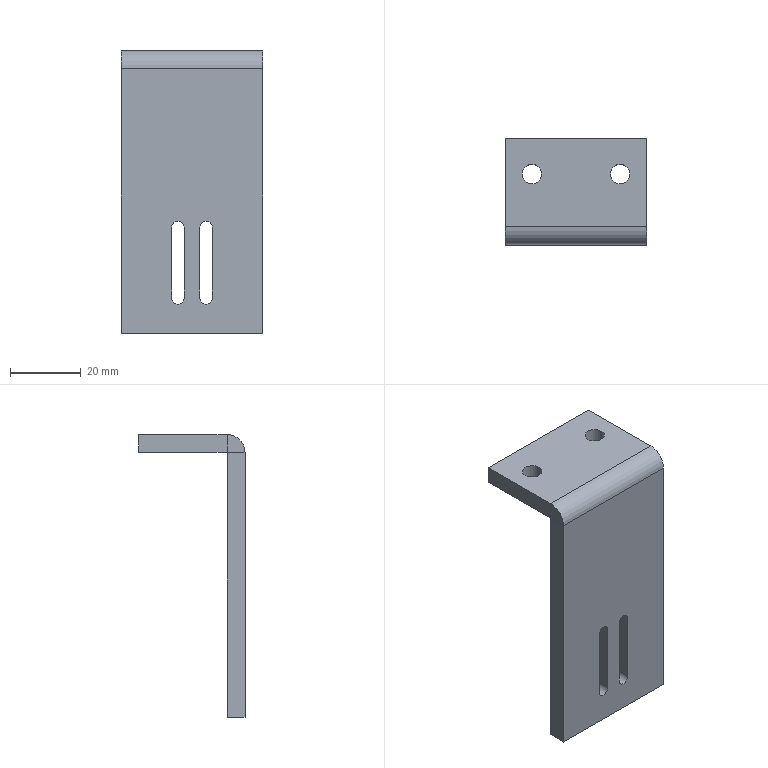Component | SolidWorks | CableChainABracket-0510-1 | 1 solid | 28 faces | box 40 x 30 x 80 mm | volume 19743 mm3 | plane 16 | cylinder 12 | commonest cylinder face diameters 3.5 x6 5.5 x4 10.2 x1 0.2 x1 | material Q235-A
STEP:
#1=COLOUR_RGB('',0.7922,0.8196,0.9333);
#2=FILL_AREA_STYLE_COLOUR('',#1);
#3=FILL_AREA_STYLE('',(#2));
#4=SURFACE_STYLE_FILL_AREA(#3);
#5=SURFACE_SIDE_STYLE('',(#4));
#6=SURFACE_STYLE_USAGE(.BOTH.,#5);
#7=PRESENTATION_STYLE_ASSIGNMENT((#6));
#8=CARTESIAN_POINT('',(-123.026,-0.772,135.295));
#9=VERTEX_POINT('',#8);
#10=CARTESIAN_POINT('',(-122.957,-0.772,135.364));
#11=VERTEX_POINT('',#10);
#12=CARTESIAN_POINT('',(-122.957,-0.772,135.295));
#13=DIRECTION('',(0.,1.,-0.));
#14=DIRECTION('',(0.,0.,-1.));
#15=AXIS2_PLACEMENT_3D('',#12,#13,#14);
#16=CIRCLE('',#15,0.0689);
#17=EDGE_CURVE('',#9,#11,#16,.T.);
#18=ORIENTED_EDGE('',*,*,#17,.T.);
#19=CARTESIAN_POINT('',(-122.957,-0.9688,135.364));
#20=VERTEX_POINT('',#19);
#21=CARTESIAN_POINT('',(-122.957,0.2123,135.364));
#22=DIRECTION('',(-0.,-1.,0.));
#23=VECTOR('',#22,39.37);
#24=LINE('',#21,#23);
#25=EDGE_CURVE('',#11,#20,#24,.T.);
#26=ORIENTED_EDGE('',*,*,#25,.T.);
#27=CARTESIAN_POINT('',(-123.026,-0.9688,135.295));
#28=VERTEX_POINT('',#27);
#29=CARTESIAN_POINT('',(-122.957,-0.9688,135.295));
#30=DIRECTION('',(-0.,-1.,0.));
#31=DIRECTION('',(0.,0.,1.));
#32=AXIS2_PLACEMENT_3D('',#29,#30,#31);
#33=CIRCLE('',#32,0.0689);
#34=EDGE_CURVE('',#20,#28,#33,.T.);
#35=ORIENTED_EDGE('',*,*,#34,.T.);
#36=CARTESIAN_POINT('',(-123.026,0.2123,135.295));
#37=DIRECTION('',(-0.,-1.,0.));
#38=VECTOR('',#37,39.37);
#39=LINE('',#36,#38);
#40=EDGE_CURVE('',#9,#28,#39,.T.);
#41=ORIENTED_EDGE('',*,*,#40,.F.);
#42=EDGE_LOOP('',(#18,#26,#35,#41));
#43=FACE_OUTER_BOUND('',#42,.T.);
#44=CARTESIAN_POINT('',(-122.957,0.2123,135.295));
#45=DIRECTION('',(-0.,-1.,0.));
#46=DIRECTION('',(0.,0.,1.));
#47=AXIS2_PLACEMENT_3D('',#44,#45,#46);
#48=CYLINDRICAL_SURFACE('',#47,0.0689);
#49=ADVANCED_FACE('',(#43),#48,.F.);
#50=CARTESIAN_POINT('',(-122.711,-0.772,135.295));
#51=VERTEX_POINT('',#50);
#52=CARTESIAN_POINT('',(-122.642,-0.772,135.364));
#53=VERTEX_POINT('',#52);
#54=CARTESIAN_POINT('',(-122.642,-0.772,135.295));
#55=DIRECTION('',(0.,1.,-0.));
#56=DIRECTION('',(0.,0.,-1.));
#57=AXIS2_PLACEMENT_3D('',#54,#55,#56);
#58=CIRCLE('',#57,0.0689);
#59=EDGE_CURVE('',#51,#53,#58,.T.);
#60=ORIENTED_EDGE('',*,*,#59,.T.);
#61=CARTESIAN_POINT('',(-122.642,-0.9688,135.364));
#62=VERTEX_POINT('',#61);
#63=CARTESIAN_POINT('',(-122.642,0.2123,135.364));
#64=DIRECTION('',(-0.,-1.,0.));
#65=VECTOR('',#64,39.37);
#66=LINE('',#63,#65);
#67=EDGE_CURVE('',#53,#62,#66,.T.);
#68=ORIENTED_EDGE('',*,*,#67,.T.);
#69=CARTESIAN_POINT('',(-122.711,-0.9688,135.295));
#70=VERTEX_POINT('',#69);
#71=CARTESIAN_POINT('',(-122.642,-0.9688,135.295));
#72=DIRECTION('',(-0.,-1.,0.));
#73=DIRECTION('',(0.,0.,1.));
#74=AXIS2_PLACEMENT_3D('',#71,#72,#73);
#75=CIRCLE('',#74,0.0689);
#76=EDGE_CURVE('',#62,#70,#75,.T.);
#77=ORIENTED_EDGE('',*,*,#76,.T.);
#78=CARTESIAN_POINT('',(-122.711,0.2123,135.295));
#79=DIRECTION('',(-0.,-1.,0.));
#80=VECTOR('',#79,39.37);
#81=LINE('',#78,#80);
#82=EDGE_CURVE('',#51,#70,#81,.T.);
#83=ORIENTED_EDGE('',*,*,#82,.F.);
#84=EDGE_LOOP('',(#60,#68,#77,#83));
#85=FACE_OUTER_BOUND('',#84,.T.);
#86=CARTESIAN_POINT('',(-122.642,0.2123,135.295));
#87=DIRECTION('',(-0.,-1.,0.));
#88=DIRECTION('',(0.,0.,1.));
#89=AXIS2_PLACEMENT_3D('',#86,#87,#88);
#90=CYLINDRICAL_SURFACE('',#89,0.0689);
#91=ADVANCED_FACE('',(#85),#90,.F.);
#92=CARTESIAN_POINT('',(-123.184,-0.1814,137.264));
#93=VERTEX_POINT('',#92);
#94=CARTESIAN_POINT('',(-123.4,-0.1814,137.264));
#95=VERTEX_POINT('',#94);
#96=CARTESIAN_POINT('',(-123.292,-0.1814,137.264));
#97=DIRECTION('',(-0.,-0.,-1.));
#98=DIRECTION('',(-1.,0.,0.));
#99=AXIS2_PLACEMENT_3D('',#96,#97,#98);
#100=CIRCLE('',#99,0.1083);
#101=EDGE_CURVE('',#93,#95,#100,.T.);
#102=ORIENTED_EDGE('',*,*,#101,.F.);
#103=CARTESIAN_POINT('',(-123.184,-0.1814,137.067));
#104=VERTEX_POINT('',#103);
#105=CARTESIAN_POINT('',(-123.184,-0.1814,137.067));
#106=DIRECTION('',(-0.,-0.,-1.));
#107=VECTOR('',#106,39.37);
#108=LINE('',#105,#107);
#109=EDGE_CURVE('',#93,#104,#108,.T.);
#110=ORIENTED_EDGE('',*,*,#109,.T.);
#111=CARTESIAN_POINT('',(-123.4,-0.1814,137.067));
#112=VERTEX_POINT('',#111);
#113=CARTESIAN_POINT('',(-123.292,-0.1814,137.067));
#114=DIRECTION('',(-0.,-0.,-1.));
#115=DIRECTION('',(-1.,0.,0.));
#116=AXIS2_PLACEMENT_3D('',#113,#114,#115);
#117=CIRCLE('',#116,0.1083);
#118=EDGE_CURVE('',#104,#112,#117,.T.);
#119=ORIENTED_EDGE('',*,*,#118,.T.);
#120=CARTESIAN_POINT('',(-123.4,-0.1814,137.067));
#121=DIRECTION('',(-0.,-0.,-1.));
#122=VECTOR('',#121,39.37);
#123=LINE('',#120,#122);
#124=EDGE_CURVE('',#95,#112,#123,.T.);
#125=ORIENTED_EDGE('',*,*,#124,.F.);
#126=EDGE_LOOP('',(#102,#110,#119,#125));
#127=FACE_OUTER_BOUND('',#126,.T.);
#128=CARTESIAN_POINT('',(-123.292,-0.1814,137.067));
#129=DIRECTION('',(-0.,-0.,-1.));
#130=DIRECTION('',(-1.,0.,0.));
#131=AXIS2_PLACEMENT_3D('',#128,#129,#130);
#132=CYLINDRICAL_SURFACE('',#131,0.1083);
#133=ADVANCED_FACE('',(#127),#132,.F.);
#134=CARTESIAN_POINT('',(-122.199,-0.1814,137.264));
#135=VERTEX_POINT('',#134);
#136=CARTESIAN_POINT('',(-122.416,-0.1814,137.264));
#137=VERTEX_POINT('',#136);
#138=CARTESIAN_POINT('',(-122.308,-0.1814,137.264));
#139=DIRECTION('',(-0.,-0.,-1.));
#140=DIRECTION('',(-1.,0.,0.));
#141=AXIS2_PLACEMENT_3D('',#138,#139,#140);
#142=CIRCLE('',#141,0.1083);
#143=EDGE_CURVE('',#135,#137,#142,.T.);
#144=ORIENTED_EDGE('',*,*,#143,.F.);
#145=CARTESIAN_POINT('',(-122.199,-0.1814,137.067));
#146=VERTEX_POINT('',#145);
#147=CARTESIAN_POINT('',(-122.199,-0.1814,137.067));
#148=DIRECTION('',(-0.,-0.,-1.));
#149=VECTOR('',#148,39.37);
#150=LINE('',#147,#149);
#151=EDGE_CURVE('',#135,#146,#150,.T.);
#152=ORIENTED_EDGE('',*,*,#151,.T.);
#153=CARTESIAN_POINT('',(-122.416,-0.1814,137.067));
#154=VERTEX_POINT('',#153);
#155=CARTESIAN_POINT('',(-122.308,-0.1814,137.067));
#156=DIRECTION('',(-0.,-0.,-1.));
#157=DIRECTION('',(-1.,0.,0.));
#158=AXIS2_PLACEMENT_3D('',#155,#156,#157);
#159=CIRCLE('',#158,0.1083);
#160=EDGE_CURVE('',#146,#154,#159,.T.);
#161=ORIENTED_EDGE('',*,*,#160,.T.);
#162=CARTESIAN_POINT('',(-122.416,-0.1814,137.067));
#163=DIRECTION('',(-0.,-0.,-1.));
#164=VECTOR('',#163,39.37);
#165=LINE('',#162,#164);
#166=EDGE_CURVE('',#137,#154,#165,.T.);
#167=ORIENTED_EDGE('',*,*,#166,.F.);
#168=EDGE_LOOP('',(#144,#152,#161,#167));
#169=FACE_OUTER_BOUND('',#168,.T.);
#170=CARTESIAN_POINT('',(-122.308,-0.1814,137.067));
#171=DIRECTION('',(-0.,-0.,-1.));
#172=DIRECTION('',(-1.,0.,0.));
#173=AXIS2_PLACEMENT_3D('',#170,#171,#172);
#174=CYLINDRICAL_SURFACE('',#173,0.1083);
#175=ADVANCED_FACE('',(#169),#174,.F.);
#176=CARTESIAN_POINT('',(-122.012,-0.772,137.063));
#177=VERTEX_POINT('',#176);
#178=CARTESIAN_POINT('',(-122.012,-0.772,134.114));
#179=VERTEX_POINT('',#178);
#180=CARTESIAN_POINT('',(-122.012,-0.772,137.264));
#181=DIRECTION('',(-0.,-0.,-1.));
#182=VECTOR('',#181,39.37);
#183=LINE('',#180,#182);
#184=EDGE_CURVE('',#177,#179,#183,.T.);
#185=ORIENTED_EDGE('',*,*,#184,.F.);
#186=CARTESIAN_POINT('',(-122.012,-0.9688,137.063));
#187=VERTEX_POINT('',#186);
#188=CARTESIAN_POINT('',(-122.012,-0.772,137.063));
#189=DIRECTION('',(-0.,-1.,0.));
#190=VECTOR('',#189,39.37);
#191=LINE('',#188,#190);
#192=EDGE_CURVE('',#177,#187,#191,.T.);
#193=ORIENTED_EDGE('',*,*,#192,.T.);
#194=CARTESIAN_POINT('',(-122.012,-0.9688,134.114));
#195=VERTEX_POINT('',#194);
#196=CARTESIAN_POINT('',(-122.012,-0.9688,137.264));
#197=DIRECTION('',(-0.,-0.,-1.));
#198=VECTOR('',#197,39.37);
#199=LINE('',#196,#198);
#200=EDGE_CURVE('',#187,#195,#199,.T.);
#201=ORIENTED_EDGE('',*,*,#200,.T.);
#202=CARTESIAN_POINT('',(-122.012,-0.9688,134.114));
#203=DIRECTION('',(0.,1.,-0.));
#204=VECTOR('',#203,39.37);
#205=LINE('',#202,#204);
#206=EDGE_CURVE('',#195,#179,#205,.T.);
#207=ORIENTED_EDGE('',*,*,#206,.T.);
#208=EDGE_LOOP('',(#185,#193,#201,#207));
#209=FACE_OUTER_BOUND('',#208,.T.);
#210=CARTESIAN_POINT('',(-122.012,-0.9688,137.264));
#211=DIRECTION('',(1.,-0.,-0.));
#212=DIRECTION('',(-0.,-0.,-1.));
#213=AXIS2_PLACEMENT_3D('',#210,#211,#212);
#214=PLANE('',#213);
#215=ADVANCED_FACE('',(#209),#214,.T.);
#216=CARTESIAN_POINT('',(-122.888,-0.9688,134.508));
#217=VERTEX_POINT('',#216);
#218=CARTESIAN_POINT('',(-122.888,-0.9688,135.295));
#219=VERTEX_POINT('',#218);
#220=CARTESIAN_POINT('',(-122.888,-0.9688,134.508));
#221=DIRECTION('',(-0.,0.,1.));
#222=VECTOR('',#221,39.37);
#223=LINE('',#220,#222);
#224=EDGE_CURVE('',#217,#219,#223,.T.);
#225=ORIENTED_EDGE('',*,*,#224,.F.);
#226=CARTESIAN_POINT('',(-123.026,-0.9688,134.508));
#227=VERTEX_POINT('',#226);
#228=CARTESIAN_POINT('',(-122.957,-0.9688,134.508));
#229=DIRECTION('',(-0.,-1.,0.));
#230=DIRECTION('',(0.,0.,1.));
#231=AXIS2_PLACEMENT_3D('',#228,#229,#230);
#232=CIRCLE('',#231,0.0689);
#233=EDGE_CURVE('',#227,#217,#232,.T.);
#234=ORIENTED_EDGE('',*,*,#233,.F.);
#235=CARTESIAN_POINT('',(-123.026,-0.9688,134.508));
#236=DIRECTION('',(0.,-0.,-1.));
#237=VECTOR('',#236,39.37);
#238=LINE('',#235,#237);
#239=EDGE_CURVE('',#28,#227,#238,.T.);
#240=ORIENTED_EDGE('',*,*,#239,.F.);
#241=ORIENTED_EDGE('',*,*,#34,.F.);
#242=CARTESIAN_POINT('',(-122.957,-0.9688,135.295));
#243=DIRECTION('',(-0.,-1.,0.));
#244=DIRECTION('',(0.,0.,1.));
#245=AXIS2_PLACEMENT_3D('',#242,#243,#244);
#246=CIRCLE('',#245,0.0689);
#247=EDGE_CURVE('',#219,#20,#246,.T.);
#248=ORIENTED_EDGE('',*,*,#247,.F.);
#249=EDGE_LOOP('',(#225,#234,#240,#241,#248));
#250=FACE_BOUND('',#249,.T.);
#251=CARTESIAN_POINT('',(-122.573,-0.9688,134.508));
#252=VERTEX_POINT('',#251);
#253=CARTESIAN_POINT('',(-122.573,-0.9688,135.295));
#254=VERTEX_POINT('',#253);
#255=CARTESIAN_POINT('',(-122.573,-0.9688,134.508));
#256=DIRECTION('',(-0.,0.,1.));
#257=VECTOR('',#256,39.37);
#258=LINE('',#255,#257);
#259=EDGE_CURVE('',#252,#254,#258,.T.);
#260=ORIENTED_EDGE('',*,*,#259,.F.);
#261=CARTESIAN_POINT('',(-122.711,-0.9688,134.508));
#262=VERTEX_POINT('',#261);
#263=CARTESIAN_POINT('',(-122.642,-0.9688,134.508));
#264=DIRECTION('',(-0.,-1.,0.));
#265=DIRECTION('',(0.,0.,1.));
#266=AXIS2_PLACEMENT_3D('',#263,#264,#265);
#267=CIRCLE('',#266,0.0689);
#268=EDGE_CURVE('',#262,#252,#267,.T.);
#269=ORIENTED_EDGE('',*,*,#268,.F.);
#270=CARTESIAN_POINT('',(-122.711,-0.9688,134.508));
#271=DIRECTION('',(0.,-0.,-1.));
#272=VECTOR('',#271,39.37);
#273=LINE('',#270,#272);
#274=EDGE_CURVE('',#70,#262,#273,.T.);
#275=ORIENTED_EDGE('',*,*,#274,.F.);
#276=ORIENTED_EDGE('',*,*,#76,.F.);
#277=CARTESIAN_POINT('',(-122.642,-0.9688,135.295));
#278=DIRECTION('',(-0.,-1.,0.));
#279=DIRECTION('',(0.,0.,1.));
#280=AXIS2_PLACEMENT_3D('',#277,#278,#279);
#281=CIRCLE('',#280,0.0689);
#282=EDGE_CURVE('',#254,#62,#281,.T.);
#283=ORIENTED_EDGE('',*,*,#282,.F.);
#284=EDGE_LOOP('',(#260,#269,#275,#276,#283));
#285=FACE_BOUND('',#284,.T.);
#286=CARTESIAN_POINT('',(-123.587,-0.9688,137.063));
#287=VERTEX_POINT('',#286);
#288=CARTESIAN_POINT('',(-122.012,-0.9688,137.063));
#289=DIRECTION('',(-1.,0.,0.));
#290=VECTOR('',#289,39.37);
#291=LINE('',#288,#290);
#292=EDGE_CURVE('',#187,#287,#291,.T.);
#293=ORIENTED_EDGE('',*,*,#292,.T.);
#294=CARTESIAN_POINT('',(-123.587,-0.9688,134.114));
#295=VERTEX_POINT('',#294);
#296=CARTESIAN_POINT('',(-123.587,-0.9688,137.264));
#297=DIRECTION('',(0.,0.,1.));
#298=VECTOR('',#297,39.37);
#299=LINE('',#296,#298);
#300=EDGE_CURVE('',#295,#287,#299,.T.);
#301=ORIENTED_EDGE('',*,*,#300,.F.);
#302=CARTESIAN_POINT('',(-122.012,-0.9688,134.114));
#303=DIRECTION('',(-1.,0.,0.));
#304=VECTOR('',#303,39.37);
#305=LINE('',#302,#304);
#306=EDGE_CURVE('',#195,#295,#305,.T.);
#307=ORIENTED_EDGE('',*,*,#306,.F.);
#308=ORIENTED_EDGE('',*,*,#200,.F.);
#309=EDGE_LOOP('',(#293,#301,#307,#308));
#310=FACE_OUTER_BOUND('',#309,.T.);
#311=CARTESIAN_POINT('',(-122.8,-0.9688,135.689));
#312=DIRECTION('',(0.,1.,-0.));
#313=DIRECTION('',(-0.,-0.,-1.));
#314=AXIS2_PLACEMENT_3D('',#311,#312,#313);
#315=PLANE('',#314);
#316=ADVANCED_FACE('',(#250,#285,#310),#315,.F.);
#317=CARTESIAN_POINT('',(-122.888,-0.772,134.508));
#318=VERTEX_POINT('',#317);
#319=CARTESIAN_POINT('',(-123.026,-0.772,134.508));
#320=VERTEX_POINT('',#319);
#321=CARTESIAN_POINT('',(-122.957,-0.772,134.508));
#322=DIRECTION('',(0.,1.,-0.));
#323=DIRECTION('',(0.,0.,-1.));
#324=AXIS2_PLACEMENT_3D('',#321,#322,#323);
#325=CIRCLE('',#324,0.0689);
#326=EDGE_CURVE('',#318,#320,#325,.T.);
#327=ORIENTED_EDGE('',*,*,#326,.F.);
#328=CARTESIAN_POINT('',(-122.888,-0.772,135.295));
#329=VERTEX_POINT('',#328);
#330=CARTESIAN_POINT('',(-122.888,-0.772,135.689));
#331=DIRECTION('',(0.,-0.,-1.));
#332=VECTOR('',#331,39.37);
#333=LINE('',#330,#332);
#334=EDGE_CURVE('',#329,#318,#333,.T.);
#335=ORIENTED_EDGE('',*,*,#334,.F.);
#336=CARTESIAN_POINT('',(-122.957,-0.772,135.295));
#337=DIRECTION('',(0.,1.,-0.));
#338=DIRECTION('',(0.,0.,-1.));
#339=AXIS2_PLACEMENT_3D('',#336,#337,#338);
#340=CIRCLE('',#339,0.0689);
#341=EDGE_CURVE('',#11,#329,#340,.T.);
#342=ORIENTED_EDGE('',*,*,#341,.F.);
#343=ORIENTED_EDGE('',*,*,#17,.F.);
#344=CARTESIAN_POINT('',(-123.026,-0.772,135.689));
#345=DIRECTION('',(-0.,0.,1.));
#346=VECTOR('',#345,39.37);
#347=LINE('',#344,#346);
#348=EDGE_CURVE('',#320,#9,#347,.T.);
#349=ORIENTED_EDGE('',*,*,#348,.F.);
#350=EDGE_LOOP('',(#327,#335,#342,#343,#349));
#351=FACE_BOUND('',#350,.T.);
#352=CARTESIAN_POINT('',(-122.573,-0.772,134.508));
#353=VERTEX_POINT('',#352);
#354=CARTESIAN_POINT('',(-122.711,-0.772,134.508));
#355=VERTEX_POINT('',#354);
#356=CARTESIAN_POINT('',(-122.642,-0.772,134.508));
#357=DIRECTION('',(0.,1.,-0.));
#358=DIRECTION('',(0.,0.,-1.));
#359=AXIS2_PLACEMENT_3D('',#356,#357,#358);
#360=CIRCLE('',#359,0.0689);
#361=EDGE_CURVE('',#353,#355,#360,.T.);
#362=ORIENTED_EDGE('',*,*,#361,.F.);
#363=CARTESIAN_POINT('',(-122.573,-0.772,135.295));
#364=VERTEX_POINT('',#363);
#365=CARTESIAN_POINT('',(-122.573,-0.772,135.689));
#366=DIRECTION('',(0.,-0.,-1.));
#367=VECTOR('',#366,39.37);
#368=LINE('',#365,#367);
#369=EDGE_CURVE('',#364,#353,#368,.T.);
#370=ORIENTED_EDGE('',*,*,#369,.F.);
#371=CARTESIAN_POINT('',(-122.642,-0.772,135.295));
#372=DIRECTION('',(0.,1.,-0.));
#373=DIRECTION('',(0.,0.,-1.));
#374=AXIS2_PLACEMENT_3D('',#371,#372,#373);
#375=CIRCLE('',#374,0.0689);
#376=EDGE_CURVE('',#53,#364,#375,.T.);
#377=ORIENTED_EDGE('',*,*,#376,.F.);
#378=ORIENTED_EDGE('',*,*,#59,.F.);
#379=CARTESIAN_POINT('',(-122.711,-0.772,135.689));
#380=DIRECTION('',(-0.,0.,1.));
#381=VECTOR('',#380,39.37);
#382=LINE('',#379,#381);
#383=EDGE_CURVE('',#355,#51,#382,.T.);
#384=ORIENTED_EDGE('',*,*,#383,.F.);
#385=EDGE_LOOP('',(#362,#370,#377,#378,#384));
#386=FACE_BOUND('',#385,.T.);
#387=CARTESIAN_POINT('',(-123.587,-0.772,134.114));
#388=VERTEX_POINT('',#387);
#389=CARTESIAN_POINT('',(-123.587,-0.772,137.063));
#390=VERTEX_POINT('',#389);
#391=CARTESIAN_POINT('',(-123.587,-0.772,137.264));
#392=DIRECTION('',(0.,0.,1.));
#393=VECTOR('',#392,39.37);
#394=LINE('',#391,#393);
#395=EDGE_CURVE('',#388,#390,#394,.T.);
#396=ORIENTED_EDGE('',*,*,#395,.T.);
#397=CARTESIAN_POINT('',(-122.012,-0.772,137.063));
#398=DIRECTION('',(-1.,0.,0.));
#399=VECTOR('',#398,39.37);
#400=LINE('',#397,#399);
#401=EDGE_CURVE('',#177,#390,#400,.T.);
#402=ORIENTED_EDGE('',*,*,#401,.F.);
#403=ORIENTED_EDGE('',*,*,#184,.T.);
#404=CARTESIAN_POINT('',(-122.012,-0.772,134.114));
#405=DIRECTION('',(-1.,0.,0.));
#406=VECTOR('',#405,39.37);
#407=LINE('',#404,#406);
#408=EDGE_CURVE('',#179,#388,#407,.T.);
#409=ORIENTED_EDGE('',*,*,#408,.T.);
#410=EDGE_LOOP('',(#396,#402,#403,#409));
#411=FACE_OUTER_BOUND('',#410,.T.);
#412=CARTESIAN_POINT('',(-122.8,-0.772,135.689));
#413=DIRECTION('',(0.,1.,-0.));
#414=DIRECTION('',(-0.,-0.,-1.));
#415=AXIS2_PLACEMENT_3D('',#412,#413,#414);
#416=PLANE('',#415);
#417=ADVANCED_FACE('',(#351,#386,#411),#416,.T.);
#418=CARTESIAN_POINT('',(-123.587,-0.772,137.063));
#419=DIRECTION('',(-0.,-1.,0.));
#420=VECTOR('',#419,39.37);
#421=LINE('',#418,#420);
#422=EDGE_CURVE('',#390,#287,#421,.T.);
#423=ORIENTED_EDGE('',*,*,#422,.F.);
#424=ORIENTED_EDGE('',*,*,#395,.F.);
#425=CARTESIAN_POINT('',(-123.587,-0.9688,134.114));
#426=DIRECTION('',(0.,1.,-0.));
#427=VECTOR('',#426,39.37);
#428=LINE('',#425,#427);
#429=EDGE_CURVE('',#295,#388,#428,.T.);
#430=ORIENTED_EDGE('',*,*,#429,.F.);
#431=ORIENTED_EDGE('',*,*,#300,.T.);
#432=EDGE_LOOP('',(#423,#424,#430,#431));
#433=FACE_OUTER_BOUND('',#432,.T.);
#434=CARTESIAN_POINT('',(-123.587,-0.9688,137.264));
#435=DIRECTION('',(-1.,0.,0.));
#436=DIRECTION('',(0.,0.,1.));
#437=AXIS2_PLACEMENT_3D('',#434,#435,#436);
#438=PLANE('',#437);
#439=ADVANCED_FACE('',(#433),#438,.T.);
#440=ORIENTED_EDGE('',*,*,#408,.F.);
#441=ORIENTED_EDGE('',*,*,#206,.F.);
#442=ORIENTED_EDGE('',*,*,#306,.T.);
#443=ORIENTED_EDGE('',*,*,#429,.T.);
#444=EDGE_LOOP('',(#440,#441,#442,#443));
#445=FACE_OUTER_BOUND('',#444,.T.);
#446=CARTESIAN_POINT('',(-122.012,-0.9688,134.114));
#447=DIRECTION('',(-0.,-0.,-1.));
#448=DIRECTION('',(-1.,0.,0.));
#449=AXIS2_PLACEMENT_3D('',#446,#447,#448);
#450=PLANE('',#449);
#451=ADVANCED_FACE('',(#445),#450,.T.);
#452=CARTESIAN_POINT('',(-123.587,-0.7681,137.067));
#453=VERTEX_POINT('',#452);
#454=CARTESIAN_POINT('',(-123.587,-0.7681,137.264));
#455=VERTEX_POINT('',#454);
#456=CARTESIAN_POINT('',(-123.587,-0.7681,137.264));
#457=DIRECTION('',(0.,0.,1.));
#458=VECTOR('',#457,39.37);
#459=LINE('',#456,#458);
#460=EDGE_CURVE('',#453,#455,#459,.T.);
#461=ORIENTED_EDGE('',*,*,#460,.F.);
#462=CARTESIAN_POINT('',(-123.587,-0.7681,137.063));
#463=DIRECTION('',(-1.,0.,0.));
#464=DIRECTION('',(0.,0.,-1.));
#465=AXIS2_PLACEMENT_3D('',#462,#463,#464);
#466=CIRCLE('',#465,0.003937);
#467=EDGE_CURVE('',#390,#453,#466,.T.);
#468=ORIENTED_EDGE('',*,*,#467,.F.);
#469=ORIENTED_EDGE('',*,*,#422,.T.);
#470=CARTESIAN_POINT('',(-123.587,-0.7681,137.063));
#471=DIRECTION('',(-1.,0.,0.));
#472=DIRECTION('',(0.,-0.,-1.));
#473=AXIS2_PLACEMENT_3D('',#470,#471,#472);
#474=CIRCLE('',#473,0.2008);
#475=EDGE_CURVE('',#287,#455,#474,.T.);
#476=ORIENTED_EDGE('',*,*,#475,.T.);
#477=EDGE_LOOP('',(#461,#468,#469,#476));
#478=FACE_OUTER_BOUND('',#477,.T.);
#479=CARTESIAN_POINT('',(-123.587,-0.7681,137.063));
#480=DIRECTION('',(-1.,0.,0.));
#481=DIRECTION('',(0.,0.,1.));
#482=AXIS2_PLACEMENT_3D('',#479,#480,#481);
#483=PLANE('',#482);
#484=ADVANCED_FACE('',(#478),#483,.T.);
#485=CARTESIAN_POINT('',(-122.012,-0.7681,137.067));
#486=VERTEX_POINT('',#485);
#487=CARTESIAN_POINT('',(-122.012,-0.7681,137.063));
#488=DIRECTION('',(1.,-0.,-0.));
#489=DIRECTION('',(0.,0.,-1.));
#490=AXIS2_PLACEMENT_3D('',#487,#488,#489);
#491=CIRCLE('',#490,0.003937);
#492=EDGE_CURVE('',#486,#177,#491,.T.);
#493=ORIENTED_EDGE('',*,*,#492,.F.);
#494=CARTESIAN_POINT('',(-122.012,-0.7681,137.264));
#495=VERTEX_POINT('',#494);
#496=CARTESIAN_POINT('',(-122.012,-0.7681,137.067));
#497=DIRECTION('',(0.,0.,1.));
#498=VECTOR('',#497,39.37);
#499=LINE('',#496,#498);
#500=EDGE_CURVE('',#486,#495,#499,.T.);
#501=ORIENTED_EDGE('',*,*,#500,.T.);
#502=CARTESIAN_POINT('',(-122.012,-0.7681,137.063));
#503=DIRECTION('',(1.,-0.,-0.));
#504=DIRECTION('',(0.,-0.,-1.));
#505=AXIS2_PLACEMENT_3D('',#502,#503,#504);
#506=CIRCLE('',#505,0.2008);
#507=EDGE_CURVE('',#495,#187,#506,.T.);
#508=ORIENTED_EDGE('',*,*,#507,.T.);
#509=ORIENTED_EDGE('',*,*,#192,.F.);
#510=EDGE_LOOP('',(#493,#501,#508,#509));
#511=FACE_OUTER_BOUND('',#510,.T.);
#512=CARTESIAN_POINT('',(-122.012,-0.7681,137.063));
#513=DIRECTION('',(-1.,0.,0.));
#514=DIRECTION('',(0.,0.,1.));
#515=AXIS2_PLACEMENT_3D('',#512,#513,#514);
#516=PLANE('',#515);
#517=ADVANCED_FACE('',(#511),#516,.F.);
#518=ORIENTED_EDGE('',*,*,#292,.F.);
#519=ORIENTED_EDGE('',*,*,#507,.F.);
#520=CARTESIAN_POINT('',(-123.587,-0.7681,137.264));
#521=DIRECTION('',(-1.,0.,0.));
#522=VECTOR('',#521,39.37);
#523=LINE('',#520,#522);
#524=EDGE_CURVE('',#495,#455,#523,.T.);
#525=ORIENTED_EDGE('',*,*,#524,.T.);
#526=ORIENTED_EDGE('',*,*,#475,.F.);
#527=EDGE_LOOP('',(#518,#519,#525,#526));
#528=FACE_OUTER_BOUND('',#527,.T.);
#529=CARTESIAN_POINT('',(-122.012,-0.7681,137.063));
#530=DIRECTION('',(1.,-0.,-0.));
#531=DIRECTION('',(0.,-0.,1.));
#532=AXIS2_PLACEMENT_3D('',#529,#530,#531);
#533=CYLINDRICAL_SURFACE('',#532,0.2008);
#534=ADVANCED_FACE('',(#528),#533,.T.);
#535=ORIENTED_EDGE('',*,*,#401,.T.);
#536=ORIENTED_EDGE('',*,*,#467,.T.);
#537=CARTESIAN_POINT('',(-123.587,-0.7681,137.067));
#538=DIRECTION('',(1.,-0.,-0.));
#539=VECTOR('',#538,39.37);
#540=LINE('',#537,#539);
#541=EDGE_CURVE('',#453,#486,#540,.T.);
#542=ORIENTED_EDGE('',*,*,#541,.T.);
#543=ORIENTED_EDGE('',*,*,#492,.T.);
#544=EDGE_LOOP('',(#535,#536,#542,#543));
#545=FACE_OUTER_BOUND('',#544,.T.);
#546=CARTESIAN_POINT('',(-122.012,-0.7681,137.063));
#547=DIRECTION('',(1.,-0.,-0.));
#548=DIRECTION('',(0.,0.,1.));
#549=AXIS2_PLACEMENT_3D('',#546,#547,#548);
#550=CYLINDRICAL_SURFACE('',#549,0.003937);
#551=ADVANCED_FACE('',(#545),#550,.F.);
#552=ORIENTED_EDGE('',*,*,#460,.T.);
#553=CARTESIAN_POINT('',(-123.587,0.2123,137.264));
#554=VERTEX_POINT('',#553);
#555=CARTESIAN_POINT('',(-123.587,-0.772,137.264));
#556=DIRECTION('',(-0.,-1.,-0.));
#557=VECTOR('',#556,39.37);
#558=LINE('',#555,#557);
#559=EDGE_CURVE('',#554,#455,#558,.T.);
#560=ORIENTED_EDGE('',*,*,#559,.F.);
#561=CARTESIAN_POINT('',(-123.587,0.2123,137.067));
#562=VERTEX_POINT('',#561);
#563=CARTESIAN_POINT('',(-123.587,0.2123,137.264));
#564=DIRECTION('',(-0.,0.,-1.));
#565=VECTOR('',#564,39.37);
#566=LINE('',#563,#565);
#567=EDGE_CURVE('',#554,#562,#566,.T.);
#568=ORIENTED_EDGE('',*,*,#567,.T.);
#569=CARTESIAN_POINT('',(-123.587,-0.772,137.067));
#570=DIRECTION('',(-0.,-1.,-0.));
#571=VECTOR('',#570,39.37);
#572=LINE('',#569,#571);
#573=EDGE_CURVE('',#562,#453,#572,.T.);
#574=ORIENTED_EDGE('',*,*,#573,.T.);
#575=EDGE_LOOP('',(#552,#560,#568,#574));
#576=FACE_OUTER_BOUND('',#575,.T.);
#577=CARTESIAN_POINT('',(-123.587,-0.772,137.264));
#578=DIRECTION('',(1.,-0.,-0.));
#579=DIRECTION('',(-0.,-0.,-1.));
#580=AXIS2_PLACEMENT_3D('',#577,#578,#579);
#581=PLANE('',#580);
#582=ADVANCED_FACE('',(#576),#581,.F.);
#583=ORIENTED_EDGE('',*,*,#500,.F.);
#584=CARTESIAN_POINT('',(-122.012,0.2123,137.067));
#585=VERTEX_POINT('',#584);
#586=CARTESIAN_POINT('',(-122.012,0.2123,137.067));
#587=DIRECTION('',(0.,1.,0.));
#588=VECTOR('',#587,39.37);
#589=LINE('',#586,#588);
#590=EDGE_CURVE('',#486,#585,#589,.T.);
#591=ORIENTED_EDGE('',*,*,#590,.T.);
#592=CARTESIAN_POINT('',(-122.012,0.2123,137.264));
#593=VERTEX_POINT('',#592);
#594=CARTESIAN_POINT('',(-122.012,0.2123,137.264));
#595=DIRECTION('',(-0.,0.,-1.));
#596=VECTOR('',#595,39.37);
#597=LINE('',#594,#596);
#598=EDGE_CURVE('',#593,#585,#597,.T.);
#599=ORIENTED_EDGE('',*,*,#598,.F.);
#600=CARTESIAN_POINT('',(-122.012,-0.772,137.264));
#601=DIRECTION('',(0.,1.,0.));
#602=VECTOR('',#601,39.37);
#603=LINE('',#600,#602);
#604=EDGE_CURVE('',#495,#593,#603,.T.);
#605=ORIENTED_EDGE('',*,*,#604,.F.);
#606=EDGE_LOOP('',(#583,#591,#599,#605));
#607=FACE_OUTER_BOUND('',#606,.T.);
#608=CARTESIAN_POINT('',(-122.012,0.2123,137.264));
#609=DIRECTION('',(-1.,0.,0.));
#610=DIRECTION('',(0.,0.,1.));
#611=AXIS2_PLACEMENT_3D('',#608,#609,#610);
#612=PLANE('',#611);
#613=ADVANCED_FACE('',(#607),#612,.F.);
#614=CARTESIAN_POINT('',(-123.292,-0.1814,137.264));
#615=DIRECTION('',(-0.,-0.,-1.));
#616=DIRECTION('',(-1.,0.,0.));
#617=AXIS2_PLACEMENT_3D('',#614,#615,#616);
#618=CIRCLE('',#617,0.1083);
#619=EDGE_CURVE('',#95,#93,#618,.T.);
#620=ORIENTED_EDGE('',*,*,#619,.T.);
#621=ORIENTED_EDGE('',*,*,#101,.T.);
#622=EDGE_LOOP('',(#620,#621));
#623=FACE_BOUND('',#622,.T.);
#624=CARTESIAN_POINT('',(-122.308,-0.1814,137.264));
#625=DIRECTION('',(-0.,-0.,-1.));
#626=DIRECTION('',(-1.,0.,0.));
#627=AXIS2_PLACEMENT_3D('',#624,#625,#626);
#628=CIRCLE('',#627,0.1083);
#629=EDGE_CURVE('',#137,#135,#628,.T.);
#630=ORIENTED_EDGE('',*,*,#629,.T.);
#631=ORIENTED_EDGE('',*,*,#143,.T.);
#632=EDGE_LOOP('',(#630,#631));
#633=FACE_BOUND('',#632,.T.);
#634=ORIENTED_EDGE('',*,*,#524,.F.);
#635=ORIENTED_EDGE('',*,*,#604,.T.);
#636=CARTESIAN_POINT('',(-122.8,0.2123,137.264));
#637=DIRECTION('',(-1.,0.,0.));
#638=VECTOR('',#637,39.37);
#639=LINE('',#636,#638);
#640=EDGE_CURVE('',#593,#554,#639,.T.);
#641=ORIENTED_EDGE('',*,*,#640,.T.);
#642=ORIENTED_EDGE('',*,*,#559,.T.);
#643=EDGE_LOOP('',(#634,#635,#641,#642));
#644=FACE_OUTER_BOUND('',#643,.T.);
#645=CARTESIAN_POINT('',(-122.8,-0.772,137.264));
#646=DIRECTION('',(-0.,0.,-1.));
#647=DIRECTION('',(-0.,-1.,-0.));
#648=AXIS2_PLACEMENT_3D('',#645,#646,#647);
#649=PLANE('',#648);
#650=ADVANCED_FACE('',(#623,#633,#644),#649,.F.);
#651=CARTESIAN_POINT('',(-123.292,-0.1814,137.067));
#652=DIRECTION('',(-0.,-0.,-1.));
#653=DIRECTION('',(-1.,0.,0.));
#654=AXIS2_PLACEMENT_3D('',#651,#652,#653);
#655=CIRCLE('',#654,0.1083);
#656=EDGE_CURVE('',#112,#104,#655,.T.);
#657=ORIENTED_EDGE('',*,*,#656,.F.);
#658=ORIENTED_EDGE('',*,*,#118,.F.);
#659=EDGE_LOOP('',(#657,#658));
#660=FACE_BOUND('',#659,.T.);
#661=CARTESIAN_POINT('',(-122.308,-0.1814,137.067));
#662=DIRECTION('',(-0.,-0.,-1.));
#663=DIRECTION('',(-1.,0.,0.));
#664=AXIS2_PLACEMENT_3D('',#661,#662,#663);
#665=CIRCLE('',#664,0.1083);
#666=EDGE_CURVE('',#154,#146,#665,.T.);
#667=ORIENTED_EDGE('',*,*,#666,.F.);
#668=ORIENTED_EDGE('',*,*,#160,.F.);
#669=EDGE_LOOP('',(#667,#668));
#670=FACE_BOUND('',#669,.T.);
#671=ORIENTED_EDGE('',*,*,#590,.F.);
#672=ORIENTED_EDGE('',*,*,#541,.F.);
#673=ORIENTED_EDGE('',*,*,#573,.F.);
#674=CARTESIAN_POINT('',(-123.587,0.2123,137.067));
#675=DIRECTION('',(-1.,0.,0.));
#676=VECTOR('',#675,39.37);
#677=LINE('',#674,#676);
#678=EDGE_CURVE('',#585,#562,#677,.T.);
#679=ORIENTED_EDGE('',*,*,#678,.F.);
#680=EDGE_LOOP('',(#671,#672,#673,#679));
#681=FACE_OUTER_BOUND('',#680,.T.);
#682=CARTESIAN_POINT('',(-122.8,-0.772,137.067));
#683=DIRECTION('',(-0.,0.,-1.));
#684=DIRECTION('',(-0.,-1.,-0.));
#685=AXIS2_PLACEMENT_3D('',#682,#683,#684);
#686=PLANE('',#685);
#687=ADVANCED_FACE('',(#660,#670,#681),#686,.T.);
#688=ORIENTED_EDGE('',*,*,#678,.T.);
#689=ORIENTED_EDGE('',*,*,#567,.F.);
#690=ORIENTED_EDGE('',*,*,#640,.F.);
#691=ORIENTED_EDGE('',*,*,#598,.T.);
#692=EDGE_LOOP('',(#688,#689,#690,#691));
#693=FACE_OUTER_BOUND('',#692,.T.);
#694=CARTESIAN_POINT('',(-123.587,0.2123,137.264));
#695=DIRECTION('',(-0.,-1.,-0.));
#696=DIRECTION('',(0.,-0.,1.));
#697=AXIS2_PLACEMENT_3D('',#694,#695,#696);
#698=PLANE('',#697);
#699=ADVANCED_FACE('',(#693),#698,.F.);
#700=ORIENTED_EDGE('',*,*,#151,.F.);
#701=ORIENTED_EDGE('',*,*,#629,.F.);
#702=ORIENTED_EDGE('',*,*,#166,.T.);
#703=ORIENTED_EDGE('',*,*,#666,.T.);
#704=EDGE_LOOP('',(#700,#701,#702,#703));
#705=FACE_OUTER_BOUND('',#704,.T.);
#706=CARTESIAN_POINT('',(-122.308,-0.1814,137.067));
#707=DIRECTION('',(-0.,-0.,-1.));
#708=DIRECTION('',(-1.,0.,0.));
#709=AXIS2_PLACEMENT_3D('',#706,#707,#708);
#710=CYLINDRICAL_SURFACE('',#709,0.1083);
#711=ADVANCED_FACE('',(#705),#710,.F.);
#712=ORIENTED_EDGE('',*,*,#109,.F.);
#713=ORIENTED_EDGE('',*,*,#619,.F.);
#714=ORIENTED_EDGE('',*,*,#124,.T.);
#715=ORIENTED_EDGE('',*,*,#656,.T.);
#716=EDGE_LOOP('',(#712,#713,#714,#715));
#717=FACE_OUTER_BOUND('',#716,.T.);
#718=CARTESIAN_POINT('',(-123.292,-0.1814,137.067));
#719=DIRECTION('',(-0.,-0.,-1.));
#720=DIRECTION('',(-1.,0.,0.));
#721=AXIS2_PLACEMENT_3D('',#718,#719,#720);
#722=CYLINDRICAL_SURFACE('',#721,0.1083);
#723=ADVANCED_FACE('',(#717),#722,.F.);
#724=ORIENTED_EDGE('',*,*,#361,.T.);
#725=CARTESIAN_POINT('',(-122.711,0.2123,134.508));
#726=DIRECTION('',(-0.,-1.,0.));
#727=VECTOR('',#726,39.37);
#728=LINE('',#725,#727);
#729=EDGE_CURVE('',#355,#262,#728,.T.);
#730=ORIENTED_EDGE('',*,*,#729,.T.);
#731=ORIENTED_EDGE('',*,*,#268,.T.);
#732=CARTESIAN_POINT('',(-122.573,0.2123,134.508));
#733=DIRECTION('',(-0.,-1.,0.));
#734=VECTOR('',#733,39.37);
#735=LINE('',#732,#734);
#736=EDGE_CURVE('',#353,#252,#735,.T.);
#737=ORIENTED_EDGE('',*,*,#736,.F.);
#738=EDGE_LOOP('',(#724,#730,#731,#737));
#739=FACE_OUTER_BOUND('',#738,.T.);
#740=CARTESIAN_POINT('',(-122.642,0.2123,134.508));
#741=DIRECTION('',(-0.,-1.,0.));
#742=DIRECTION('',(0.,0.,1.));
#743=AXIS2_PLACEMENT_3D('',#740,#741,#742);
#744=CYLINDRICAL_SURFACE('',#743,0.0689);
#745=ADVANCED_FACE('',(#739),#744,.F.);
#746=ORIENTED_EDGE('',*,*,#383,.T.);
#747=ORIENTED_EDGE('',*,*,#82,.T.);
#748=ORIENTED_EDGE('',*,*,#274,.T.);
#749=ORIENTED_EDGE('',*,*,#729,.F.);
#750=EDGE_LOOP('',(#746,#747,#748,#749));
#751=FACE_OUTER_BOUND('',#750,.T.);
#752=CARTESIAN_POINT('',(-122.711,0.2123,134.508));
#753=DIRECTION('',(-1.,0.,-0.));
#754=DIRECTION('',(-0.,0.,1.));
#755=AXIS2_PLACEMENT_3D('',#752,#753,#754);
#756=PLANE('',#755);
#757=ADVANCED_FACE('',(#751),#756,.F.);
#758=ORIENTED_EDGE('',*,*,#67,.F.);
#759=ORIENTED_EDGE('',*,*,#376,.T.);
#760=CARTESIAN_POINT('',(-122.573,0.2123,135.295));
#761=DIRECTION('',(-0.,-1.,0.));
#762=VECTOR('',#761,39.37);
#763=LINE('',#760,#762);
#764=EDGE_CURVE('',#364,#254,#763,.T.);
#765=ORIENTED_EDGE('',*,*,#764,.T.);
#766=ORIENTED_EDGE('',*,*,#282,.T.);
#767=EDGE_LOOP('',(#758,#759,#765,#766));
#768=FACE_OUTER_BOUND('',#767,.T.);
#769=CARTESIAN_POINT('',(-122.642,0.2123,135.295));
#770=DIRECTION('',(-0.,-1.,0.));
#771=DIRECTION('',(0.,0.,1.));
#772=AXIS2_PLACEMENT_3D('',#769,#770,#771);
#773=CYLINDRICAL_SURFACE('',#772,0.0689);
#774=ADVANCED_FACE('',(#768),#773,.F.);
#775=ORIENTED_EDGE('',*,*,#369,.T.);
#776=ORIENTED_EDGE('',*,*,#736,.T.);
#777=ORIENTED_EDGE('',*,*,#259,.T.);
#778=ORIENTED_EDGE('',*,*,#764,.F.);
#779=EDGE_LOOP('',(#775,#776,#777,#778));
#780=FACE_OUTER_BOUND('',#779,.T.);
#781=CARTESIAN_POINT('',(-122.573,0.2123,134.508));
#782=DIRECTION('',(1.,-0.,0.));
#783=DIRECTION('',(0.,-0.,-1.));
#784=AXIS2_PLACEMENT_3D('',#781,#782,#783);
#785=PLANE('',#784);
#786=ADVANCED_FACE('',(#780),#785,.F.);
#787=ORIENTED_EDGE('',*,*,#326,.T.);
#788=CARTESIAN_POINT('',(-123.026,0.2123,134.508));
#789=DIRECTION('',(-0.,-1.,0.));
#790=VECTOR('',#789,39.37);
#791=LINE('',#788,#790);
#792=EDGE_CURVE('',#320,#227,#791,.T.);
#793=ORIENTED_EDGE('',*,*,#792,.T.);
#794=ORIENTED_EDGE('',*,*,#233,.T.);
#795=CARTESIAN_POINT('',(-122.888,0.2123,134.508));
#796=DIRECTION('',(-0.,-1.,0.));
#797=VECTOR('',#796,39.37);
#798=LINE('',#795,#797);
#799=EDGE_CURVE('',#318,#217,#798,.T.);
#800=ORIENTED_EDGE('',*,*,#799,.F.);
#801=EDGE_LOOP('',(#787,#793,#794,#800));
#802=FACE_OUTER_BOUND('',#801,.T.);
#803=CARTESIAN_POINT('',(-122.957,0.2123,134.508));
#804=DIRECTION('',(-0.,-1.,0.));
#805=DIRECTION('',(0.,0.,1.));
#806=AXIS2_PLACEMENT_3D('',#803,#804,#805);
#807=CYLINDRICAL_SURFACE('',#806,0.0689);
#808=ADVANCED_FACE('',(#802),#807,.F.);
#809=ORIENTED_EDGE('',*,*,#348,.T.);
#810=ORIENTED_EDGE('',*,*,#40,.T.);
#811=ORIENTED_EDGE('',*,*,#239,.T.);
#812=ORIENTED_EDGE('',*,*,#792,.F.);
#813=EDGE_LOOP('',(#809,#810,#811,#812));
#814=FACE_OUTER_BOUND('',#813,.T.);
#815=CARTESIAN_POINT('',(-123.026,0.2123,134.508));
#816=DIRECTION('',(-1.,0.,-0.));
#817=DIRECTION('',(-0.,0.,1.));
#818=AXIS2_PLACEMENT_3D('',#815,#816,#817);
#819=PLANE('',#818);
#820=ADVANCED_FACE('',(#814),#819,.F.);
#821=ORIENTED_EDGE('',*,*,#25,.F.);
#822=ORIENTED_EDGE('',*,*,#341,.T.);
#823=CARTESIAN_POINT('',(-122.888,0.2123,135.295));
#824=DIRECTION('',(-0.,-1.,0.));
#825=VECTOR('',#824,39.37);
#826=LINE('',#823,#825);
#827=EDGE_CURVE('',#329,#219,#826,.T.);
#828=ORIENTED_EDGE('',*,*,#827,.T.);
#829=ORIENTED_EDGE('',*,*,#247,.T.);
#830=EDGE_LOOP('',(#821,#822,#828,#829));
#831=FACE_OUTER_BOUND('',#830,.T.);
#832=CARTESIAN_POINT('',(-122.957,0.2123,135.295));
#833=DIRECTION('',(-0.,-1.,0.));
#834=DIRECTION('',(0.,0.,1.));
#835=AXIS2_PLACEMENT_3D('',#832,#833,#834);
#836=CYLINDRICAL_SURFACE('',#835,0.0689);
#837=ADVANCED_FACE('',(#831),#836,.F.);
#838=ORIENTED_EDGE('',*,*,#334,.T.);
#839=ORIENTED_EDGE('',*,*,#799,.T.);
#840=ORIENTED_EDGE('',*,*,#224,.T.);
#841=ORIENTED_EDGE('',*,*,#827,.F.);
#842=EDGE_LOOP('',(#838,#839,#840,#841));
#843=FACE_OUTER_BOUND('',#842,.T.);
#844=CARTESIAN_POINT('',(-122.888,0.2123,134.508));
#845=DIRECTION('',(1.,-0.,0.));
#846=DIRECTION('',(0.,-0.,-1.));
#847=AXIS2_PLACEMENT_3D('',#844,#845,#846);
#848=PLANE('',#847);
#849=ADVANCED_FACE('',(#843),#848,.F.);
#850=CLOSED_SHELL('',(#49,#91,#133,#175,#215,#316,#417,#439,#451,#484,#517,#534,#551,#582,#613,#650,#687,#699,#711,#723,#745,#757,#774,#786,#808,#820,#837,#849));
#851=MANIFOLD_SOLID_BREP('',#850);
#852=STYLED_ITEM('',(#7),#851);
#853=(LENGTH_UNIT()NAMED_UNIT(*)SI_UNIT($,.METRE.));
#854=LENGTH_MEASURE_WITH_UNIT(LENGTH_MEASURE(0.0254),#853);
#855=DIMENSIONAL_EXPONENTS(1.,0.,0.,0.,0.,0.,0.);
#856=(CONVERSION_BASED_UNIT('',#854)LENGTH_UNIT()NAMED_UNIT(#855));
#857=UNCERTAINTY_MEASURE_WITH_UNIT(LENGTH_MEASURE(0.00001),#856,'','');
#858=(NAMED_UNIT(*)PLANE_ANGLE_UNIT()SI_UNIT($,.RADIAN.));
#859=(NAMED_UNIT(*)SI_UNIT($,.STERADIAN.)SOLID_ANGLE_UNIT());
#860=(GEOMETRIC_REPRESENTATION_CONTEXT(3)GLOBAL_UNCERTAINTY_ASSIGNED_CONTEXT((#857))GLOBAL_UNIT_ASSIGNED_CONTEXT((#856,#858,#859))REPRESENTATION_CONTEXT('',''));
#861=MECHANICAL_DESIGN_GEOMETRIC_PRESENTATION_REPRESENTATION('',(#852),#860);
#862=PRESENTATION_LAYER_ASSIGNMENT('','',(#852));
#863=CARTESIAN_POINT('',(0.,0.,0.));
#864=DIRECTION('',(0.,0.,1.));
#865=DIRECTION('',(1.,0.,0.));
#866=AXIS2_PLACEMENT_3D('',#863,#864,#865);
#867=(LENGTH_UNIT()NAMED_UNIT(*)SI_UNIT($,.METRE.));
#868=LENGTH_MEASURE_WITH_UNIT(LENGTH_MEASURE(0.0254),#867);
#869=DIMENSIONAL_EXPONENTS(1.,0.,0.,0.,0.,0.,0.);
#870=(CONVERSION_BASED_UNIT('',#868)LENGTH_UNIT()NAMED_UNIT(#869));
#871=UNCERTAINTY_MEASURE_WITH_UNIT(LENGTH_MEASURE(0.00001),#870,'','');
#872=(NAMED_UNIT(*)PLANE_ANGLE_UNIT()SI_UNIT($,.RADIAN.));
#873=(NAMED_UNIT(*)SI_UNIT($,.STERADIAN.)SOLID_ANGLE_UNIT());
#874=(GEOMETRIC_REPRESENTATION_CONTEXT(3)GLOBAL_UNCERTAINTY_ASSIGNED_CONTEXT((#871))GLOBAL_UNIT_ASSIGNED_CONTEXT((#870,#872,#873))REPRESENTATION_CONTEXT('',''));
#875=ADVANCED_BREP_SHAPE_REPRESENTATION('',(#851,#866),#874);